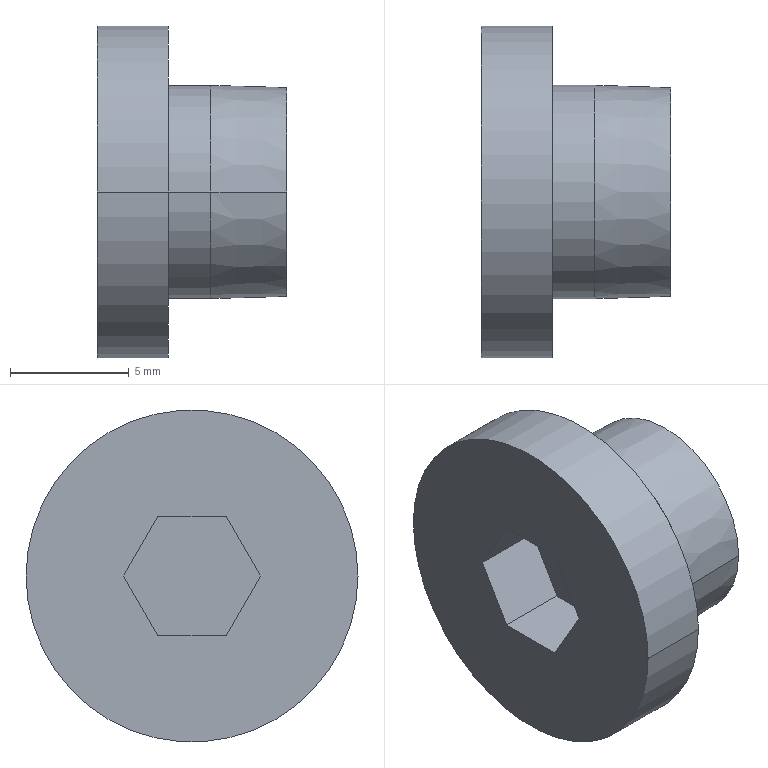Component | SolidWorks | LeverHydraulicRod22-6_Part-2 | 1 solid | 16 faces | box 8 x 14 x 14 mm | volume 710 mm3 | plane 10 | cylinder 4 | cone 2 | commonest cylinder face diameters 9 x2 14 x2
STEP:
#1=COLOUR_RGB('',0.7922,0.8196,0.9333);
#2=FILL_AREA_STYLE_COLOUR('',#1);
#3=FILL_AREA_STYLE('',(#2));
#4=SURFACE_STYLE_FILL_AREA(#3);
#5=SURFACE_SIDE_STYLE('',(#4));
#6=SURFACE_STYLE_USAGE(.BOTH.,#5);
#7=PRESENTATION_STYLE_ASSIGNMENT((#6));
#8=CARTESIAN_POINT('',(-3.607,3.128,3.307));
#9=VERTEX_POINT('',#8);
#10=CARTESIAN_POINT('',(-3.607,2.781,3.307));
#11=VERTEX_POINT('',#10);
#12=CARTESIAN_POINT('',(-3.607,2.955,3.307));
#13=DIRECTION('',(-1.,-0.,0.));
#14=DIRECTION('',(0.,-1.,0.));
#15=AXIS2_PLACEMENT_3D('',#12,#13,#14);
#16=CIRCLE('',#15,0.1732);
#17=EDGE_CURVE('',#9,#11,#16,.T.);
#18=ORIENTED_EDGE('',*,*,#17,.T.);
#19=CARTESIAN_POINT('',(-3.733,2.777,3.307));
#20=VERTEX_POINT('',#19);
#21=CARTESIAN_POINT('',(-3.745,2.777,3.307));
#22=DIRECTION('',(-0.9995,-0.0312,-0.));
#23=VECTOR('',#22,39.37);
#24=LINE('',#21,#23);
#25=EDGE_CURVE('',#11,#20,#24,.T.);
#26=ORIENTED_EDGE('',*,*,#25,.T.);
#27=CARTESIAN_POINT('',(-3.733,3.132,3.307));
#28=VERTEX_POINT('',#27);
#29=CARTESIAN_POINT('',(-3.733,2.955,3.307));
#30=DIRECTION('',(1.,0.,-0.));
#31=DIRECTION('',(0.,1.,0.));
#32=AXIS2_PLACEMENT_3D('',#29,#30,#31);
#33=CIRCLE('',#32,0.1772);
#34=EDGE_CURVE('',#20,#28,#33,.T.);
#35=ORIENTED_EDGE('',*,*,#34,.T.);
#36=CARTESIAN_POINT('',(-3.745,3.132,3.307));
#37=DIRECTION('',(-0.9995,0.0312,0.));
#38=VECTOR('',#37,39.37);
#39=LINE('',#36,#38);
#40=EDGE_CURVE('',#9,#28,#39,.T.);
#41=ORIENTED_EDGE('',*,*,#40,.F.);
#42=EDGE_LOOP('',(#18,#26,#35,#41));
#43=FACE_OUTER_BOUND('',#42,.T.);
#44=CARTESIAN_POINT('',(-3.745,2.955,3.307));
#45=DIRECTION('',(-1.,-0.,0.));
#46=DIRECTION('',(0.,1.,0.));
#47=AXIS2_PLACEMENT_3D('',#44,#45,#46);
#48=CONICAL_SURFACE('',#47,0.1775,0.03121);
#49=ADVANCED_FACE('',(#43),#48,.T.);
#50=ORIENTED_EDGE('',*,*,#34,.F.);
#51=CARTESIAN_POINT('',(-3.804,2.777,3.307));
#52=VERTEX_POINT('',#51);
#53=CARTESIAN_POINT('',(-3.607,2.777,3.307));
#54=DIRECTION('',(-1.,-0.,0.));
#55=VECTOR('',#54,39.37);
#56=LINE('',#53,#55);
#57=EDGE_CURVE('',#20,#52,#56,.T.);
#58=ORIENTED_EDGE('',*,*,#57,.T.);
#59=CARTESIAN_POINT('',(-3.804,3.132,3.307));
#60=VERTEX_POINT('',#59);
#61=CARTESIAN_POINT('',(-3.804,2.955,3.307));
#62=DIRECTION('',(1.,0.,-0.));
#63=DIRECTION('',(0.,1.,0.));
#64=AXIS2_PLACEMENT_3D('',#61,#62,#63);
#65=CIRCLE('',#64,0.1772);
#66=EDGE_CURVE('',#52,#60,#65,.T.);
#67=ORIENTED_EDGE('',*,*,#66,.T.);
#68=CARTESIAN_POINT('',(-3.607,3.132,3.307));
#69=DIRECTION('',(-1.,-0.,0.));
#70=VECTOR('',#69,39.37);
#71=LINE('',#68,#70);
#72=EDGE_CURVE('',#28,#60,#71,.T.);
#73=ORIENTED_EDGE('',*,*,#72,.F.);
#74=EDGE_LOOP('',(#50,#58,#67,#73));
#75=FACE_OUTER_BOUND('',#74,.T.);
#76=CARTESIAN_POINT('',(-3.607,2.955,3.307));
#77=DIRECTION('',(-1.,-0.,0.));
#78=DIRECTION('',(0.,1.,0.));
#79=AXIS2_PLACEMENT_3D('',#76,#77,#78);
#80=CYLINDRICAL_SURFACE('',#79,0.1772);
#81=ADVANCED_FACE('',(#75),#80,.T.);
#82=CARTESIAN_POINT('',(-3.922,3.23,3.307));
#83=VERTEX_POINT('',#82);
#84=CARTESIAN_POINT('',(-3.922,2.679,3.307));
#85=VERTEX_POINT('',#84);
#86=CARTESIAN_POINT('',(-3.922,2.955,3.307));
#87=DIRECTION('',(-1.,-0.,0.));
#88=DIRECTION('',(0.,1.,0.));
#89=AXIS2_PLACEMENT_3D('',#86,#87,#88);
#90=CIRCLE('',#89,0.2756);
#91=EDGE_CURVE('',#83,#85,#90,.T.);
#92=ORIENTED_EDGE('',*,*,#91,.F.);
#93=CARTESIAN_POINT('',(-3.804,3.23,3.307));
#94=VERTEX_POINT('',#93);
#95=CARTESIAN_POINT('',(-3.922,3.23,3.307));
#96=DIRECTION('',(1.,0.,-0.));
#97=VECTOR('',#96,39.37);
#98=LINE('',#95,#97);
#99=EDGE_CURVE('',#83,#94,#98,.T.);
#100=ORIENTED_EDGE('',*,*,#99,.T.);
#101=CARTESIAN_POINT('',(-3.804,2.679,3.307));
#102=VERTEX_POINT('',#101);
#103=CARTESIAN_POINT('',(-3.804,2.955,3.307));
#104=DIRECTION('',(-1.,-0.,0.));
#105=DIRECTION('',(0.,1.,0.));
#106=AXIS2_PLACEMENT_3D('',#103,#104,#105);
#107=CIRCLE('',#106,0.2756);
#108=EDGE_CURVE('',#94,#102,#107,.T.);
#109=ORIENTED_EDGE('',*,*,#108,.T.);
#110=CARTESIAN_POINT('',(-3.922,2.679,3.307));
#111=DIRECTION('',(1.,0.,-0.));
#112=VECTOR('',#111,39.37);
#113=LINE('',#110,#112);
#114=EDGE_CURVE('',#85,#102,#113,.T.);
#115=ORIENTED_EDGE('',*,*,#114,.F.);
#116=EDGE_LOOP('',(#92,#100,#109,#115));
#117=FACE_OUTER_BOUND('',#116,.T.);
#118=CARTESIAN_POINT('',(-3.922,2.955,3.307));
#119=DIRECTION('',(1.,0.,-0.));
#120=DIRECTION('',(0.,-1.,0.));
#121=AXIS2_PLACEMENT_3D('',#118,#119,#120);
#122=CYLINDRICAL_SURFACE('',#121,0.2756);
#123=ADVANCED_FACE('',(#117),#122,.T.);
#124=CARTESIAN_POINT('',(-3.804,2.898,3.406));
#125=VERTEX_POINT('',#124);
#126=CARTESIAN_POINT('',(-3.804,3.011,3.406));
#127=VERTEX_POINT('',#126);
#128=CARTESIAN_POINT('',(-3.804,2.898,3.406));
#129=DIRECTION('',(-0.,1.,0.));
#130=VECTOR('',#129,39.37);
#131=LINE('',#128,#130);
#132=EDGE_CURVE('',#125,#127,#131,.T.);
#133=ORIENTED_EDGE('',*,*,#132,.T.);
#134=CARTESIAN_POINT('',(-3.804,3.068,3.307));
#135=VERTEX_POINT('',#134);
#136=CARTESIAN_POINT('',(-3.804,3.011,3.406));
#137=DIRECTION('',(-0.,0.5,-0.866));
#138=VECTOR('',#137,39.37);
#139=LINE('',#136,#138);
#140=EDGE_CURVE('',#127,#135,#139,.T.);
#141=ORIENTED_EDGE('',*,*,#140,.T.);
#142=CARTESIAN_POINT('',(-3.804,3.011,3.209));
#143=VERTEX_POINT('',#142);
#144=CARTESIAN_POINT('',(-3.804,3.068,3.307));
#145=DIRECTION('',(-0.,-0.5,-0.866));
#146=VECTOR('',#145,39.37);
#147=LINE('',#144,#146);
#148=EDGE_CURVE('',#135,#143,#147,.T.);
#149=ORIENTED_EDGE('',*,*,#148,.T.);
#150=CARTESIAN_POINT('',(-3.804,2.898,3.209));
#151=VERTEX_POINT('',#150);
#152=CARTESIAN_POINT('',(-3.804,3.011,3.209));
#153=DIRECTION('',(0.,-1.,-0.));
#154=VECTOR('',#153,39.37);
#155=LINE('',#152,#154);
#156=EDGE_CURVE('',#143,#151,#155,.T.);
#157=ORIENTED_EDGE('',*,*,#156,.T.);
#158=CARTESIAN_POINT('',(-3.804,2.841,3.307));
#159=VERTEX_POINT('',#158);
#160=CARTESIAN_POINT('',(-3.804,2.898,3.209));
#161=DIRECTION('',(0.,-0.5,0.866));
#162=VECTOR('',#161,39.37);
#163=LINE('',#160,#162);
#164=EDGE_CURVE('',#151,#159,#163,.T.);
#165=ORIENTED_EDGE('',*,*,#164,.T.);
#166=CARTESIAN_POINT('',(-3.804,2.841,3.307));
#167=DIRECTION('',(0.,0.5,0.866));
#168=VECTOR('',#167,39.37);
#169=LINE('',#166,#168);
#170=EDGE_CURVE('',#159,#125,#169,.T.);
#171=ORIENTED_EDGE('',*,*,#170,.T.);
#172=EDGE_LOOP('',(#133,#141,#149,#157,#165,#171));
#173=FACE_OUTER_BOUND('',#172,.T.);
#174=CARTESIAN_POINT('',(-3.804,2.955,3.307));
#175=DIRECTION('',(-1.,-0.,0.));
#176=DIRECTION('',(-0.,1.,0.));
#177=AXIS2_PLACEMENT_3D('',#174,#175,#176);
#178=PLANE('',#177);
#179=ADVANCED_FACE('',(#173),#178,.T.);
#180=CARTESIAN_POINT('',(-3.922,3.011,3.406));
#181=VERTEX_POINT('',#180);
#182=CARTESIAN_POINT('',(-3.922,3.068,3.307));
#183=VERTEX_POINT('',#182);
#184=CARTESIAN_POINT('',(-3.922,3.011,3.406));
#185=DIRECTION('',(-0.,0.5,-0.866));
#186=VECTOR('',#185,39.37);
#187=LINE('',#184,#186);
#188=EDGE_CURVE('',#181,#183,#187,.T.);
#189=ORIENTED_EDGE('',*,*,#188,.T.);
#190=CARTESIAN_POINT('',(-3.804,3.068,3.307));
#191=DIRECTION('',(-1.,-0.,0.));
#192=VECTOR('',#191,39.37);
#193=LINE('',#190,#192);
#194=EDGE_CURVE('',#135,#183,#193,.T.);
#195=ORIENTED_EDGE('',*,*,#194,.F.);
#196=ORIENTED_EDGE('',*,*,#140,.F.);
#197=CARTESIAN_POINT('',(-3.804,3.011,3.406));
#198=DIRECTION('',(-1.,-0.,0.));
#199=VECTOR('',#198,39.37);
#200=LINE('',#197,#199);
#201=EDGE_CURVE('',#127,#181,#200,.T.);
#202=ORIENTED_EDGE('',*,*,#201,.T.);
#203=EDGE_LOOP('',(#189,#195,#196,#202));
#204=FACE_OUTER_BOUND('',#203,.T.);
#205=CARTESIAN_POINT('',(-3.804,3.011,3.406));
#206=DIRECTION('',(-0.,0.866,0.5));
#207=DIRECTION('',(1.,0.,-0.));
#208=AXIS2_PLACEMENT_3D('',#205,#206,#207);
#209=PLANE('',#208);
#210=ADVANCED_FACE('',(#204),#209,.F.);
#211=CARTESIAN_POINT('',(-3.922,3.011,3.209));
#212=VERTEX_POINT('',#211);
#213=CARTESIAN_POINT('',(-3.922,3.068,3.307));
#214=DIRECTION('',(-0.,-0.5,-0.866));
#215=VECTOR('',#214,39.37);
#216=LINE('',#213,#215);
#217=EDGE_CURVE('',#183,#212,#216,.T.);
#218=ORIENTED_EDGE('',*,*,#217,.T.);
#219=CARTESIAN_POINT('',(-3.804,3.011,3.209));
#220=DIRECTION('',(-1.,-0.,0.));
#221=VECTOR('',#220,39.37);
#222=LINE('',#219,#221);
#223=EDGE_CURVE('',#143,#212,#222,.T.);
#224=ORIENTED_EDGE('',*,*,#223,.F.);
#225=ORIENTED_EDGE('',*,*,#148,.F.);
#226=ORIENTED_EDGE('',*,*,#194,.T.);
#227=EDGE_LOOP('',(#218,#224,#225,#226));
#228=FACE_OUTER_BOUND('',#227,.T.);
#229=CARTESIAN_POINT('',(-3.804,3.068,3.307));
#230=DIRECTION('',(-0.,0.866,-0.5));
#231=DIRECTION('',(1.,0.,-0.));
#232=AXIS2_PLACEMENT_3D('',#229,#230,#231);
#233=PLANE('',#232);
#234=ADVANCED_FACE('',(#228),#233,.F.);
#235=CARTESIAN_POINT('',(-3.922,2.898,3.209));
#236=VERTEX_POINT('',#235);
#237=CARTESIAN_POINT('',(-3.922,3.011,3.209));
#238=DIRECTION('',(0.,-1.,-0.));
#239=VECTOR('',#238,39.37);
#240=LINE('',#237,#239);
#241=EDGE_CURVE('',#212,#236,#240,.T.);
#242=ORIENTED_EDGE('',*,*,#241,.T.);
#243=CARTESIAN_POINT('',(-3.804,2.898,3.209));
#244=DIRECTION('',(-1.,-0.,0.));
#245=VECTOR('',#244,39.37);
#246=LINE('',#243,#245);
#247=EDGE_CURVE('',#151,#236,#246,.T.);
#248=ORIENTED_EDGE('',*,*,#247,.F.);
#249=ORIENTED_EDGE('',*,*,#156,.F.);
#250=ORIENTED_EDGE('',*,*,#223,.T.);
#251=EDGE_LOOP('',(#242,#248,#249,#250));
#252=FACE_OUTER_BOUND('',#251,.T.);
#253=CARTESIAN_POINT('',(-3.804,3.011,3.209));
#254=DIRECTION('',(-0.,0.,-1.));
#255=DIRECTION('',(-0.,1.,0.));
#256=AXIS2_PLACEMENT_3D('',#253,#254,#255);
#257=PLANE('',#256);
#258=ADVANCED_FACE('',(#252),#257,.F.);
#259=CARTESIAN_POINT('',(-3.922,2.841,3.307));
#260=VERTEX_POINT('',#259);
#261=CARTESIAN_POINT('',(-3.922,2.898,3.209));
#262=DIRECTION('',(0.,-0.5,0.866));
#263=VECTOR('',#262,39.37);
#264=LINE('',#261,#263);
#265=EDGE_CURVE('',#236,#260,#264,.T.);
#266=ORIENTED_EDGE('',*,*,#265,.T.);
#267=CARTESIAN_POINT('',(-3.804,2.841,3.307));
#268=DIRECTION('',(-1.,-0.,0.));
#269=VECTOR('',#268,39.37);
#270=LINE('',#267,#269);
#271=EDGE_CURVE('',#159,#260,#270,.T.);
#272=ORIENTED_EDGE('',*,*,#271,.F.);
#273=ORIENTED_EDGE('',*,*,#164,.F.);
#274=ORIENTED_EDGE('',*,*,#247,.T.);
#275=EDGE_LOOP('',(#266,#272,#273,#274));
#276=FACE_OUTER_BOUND('',#275,.T.);
#277=CARTESIAN_POINT('',(-3.804,2.898,3.209));
#278=DIRECTION('',(0.,-0.866,-0.5));
#279=DIRECTION('',(-1.,-0.,0.));
#280=AXIS2_PLACEMENT_3D('',#277,#278,#279);
#281=PLANE('',#280);
#282=ADVANCED_FACE('',(#276),#281,.F.);
#283=CARTESIAN_POINT('',(-3.922,2.898,3.406));
#284=VERTEX_POINT('',#283);
#285=CARTESIAN_POINT('',(-3.922,2.841,3.307));
#286=DIRECTION('',(0.,0.5,0.866));
#287=VECTOR('',#286,39.37);
#288=LINE('',#285,#287);
#289=EDGE_CURVE('',#260,#284,#288,.T.);
#290=ORIENTED_EDGE('',*,*,#289,.T.);
#291=CARTESIAN_POINT('',(-3.804,2.898,3.406));
#292=DIRECTION('',(-1.,-0.,0.));
#293=VECTOR('',#292,39.37);
#294=LINE('',#291,#293);
#295=EDGE_CURVE('',#125,#284,#294,.T.);
#296=ORIENTED_EDGE('',*,*,#295,.F.);
#297=ORIENTED_EDGE('',*,*,#170,.F.);
#298=ORIENTED_EDGE('',*,*,#271,.T.);
#299=EDGE_LOOP('',(#290,#296,#297,#298));
#300=FACE_OUTER_BOUND('',#299,.T.);
#301=CARTESIAN_POINT('',(-3.804,2.841,3.307));
#302=DIRECTION('',(0.,-0.866,0.5));
#303=DIRECTION('',(-0.,-0.5,-0.866));
#304=AXIS2_PLACEMENT_3D('',#301,#302,#303);
#305=PLANE('',#304);
#306=ADVANCED_FACE('',(#300),#305,.F.);
#307=CARTESIAN_POINT('',(-3.922,2.898,3.406));
#308=DIRECTION('',(-0.,1.,0.));
#309=VECTOR('',#308,39.37);
#310=LINE('',#307,#309);
#311=EDGE_CURVE('',#284,#181,#310,.T.);
#312=ORIENTED_EDGE('',*,*,#311,.T.);
#313=ORIENTED_EDGE('',*,*,#201,.F.);
#314=ORIENTED_EDGE('',*,*,#132,.F.);
#315=ORIENTED_EDGE('',*,*,#295,.T.);
#316=EDGE_LOOP('',(#312,#313,#314,#315));
#317=FACE_OUTER_BOUND('',#316,.T.);
#318=CARTESIAN_POINT('',(-3.804,2.898,3.406));
#319=DIRECTION('',(0.,-0.,1.));
#320=DIRECTION('',(1.,0.,-0.));
#321=AXIS2_PLACEMENT_3D('',#318,#319,#320);
#322=PLANE('',#321);
#323=ADVANCED_FACE('',(#317),#322,.F.);
#324=ORIENTED_EDGE('',*,*,#311,.F.);
#325=ORIENTED_EDGE('',*,*,#289,.F.);
#326=ORIENTED_EDGE('',*,*,#265,.F.);
#327=ORIENTED_EDGE('',*,*,#241,.F.);
#328=ORIENTED_EDGE('',*,*,#217,.F.);
#329=ORIENTED_EDGE('',*,*,#188,.F.);
#330=EDGE_LOOP('',(#324,#325,#326,#327,#328,#329));
#331=FACE_BOUND('',#330,.T.);
#332=CARTESIAN_POINT('',(-3.922,2.955,3.307));
#333=DIRECTION('',(-1.,-0.,0.));
#334=DIRECTION('',(0.,1.,0.));
#335=AXIS2_PLACEMENT_3D('',#332,#333,#334);
#336=CIRCLE('',#335,0.2756);
#337=EDGE_CURVE('',#85,#83,#336,.T.);
#338=ORIENTED_EDGE('',*,*,#337,.T.);
#339=ORIENTED_EDGE('',*,*,#91,.T.);
#340=EDGE_LOOP('',(#338,#339));
#341=FACE_OUTER_BOUND('',#340,.T.);
#342=CARTESIAN_POINT('',(-3.922,2.955,3.307));
#343=DIRECTION('',(-1.,-0.,0.));
#344=DIRECTION('',(-0.,1.,0.));
#345=AXIS2_PLACEMENT_3D('',#342,#343,#344);
#346=PLANE('',#345);
#347=ADVANCED_FACE('',(#331,#341),#346,.T.);
#348=CARTESIAN_POINT('',(-3.804,2.955,3.307));
#349=DIRECTION('',(1.,0.,-0.));
#350=DIRECTION('',(0.,1.,0.));
#351=AXIS2_PLACEMENT_3D('',#348,#349,#350);
#352=CIRCLE('',#351,0.1772);
#353=EDGE_CURVE('',#60,#52,#352,.T.);
#354=ORIENTED_EDGE('',*,*,#353,.F.);
#355=ORIENTED_EDGE('',*,*,#66,.F.);
#356=EDGE_LOOP('',(#354,#355));
#357=FACE_BOUND('',#356,.T.);
#358=CARTESIAN_POINT('',(-3.804,2.955,3.307));
#359=DIRECTION('',(-1.,-0.,0.));
#360=DIRECTION('',(0.,1.,0.));
#361=AXIS2_PLACEMENT_3D('',#358,#359,#360);
#362=CIRCLE('',#361,0.2756);
#363=EDGE_CURVE('',#102,#94,#362,.T.);
#364=ORIENTED_EDGE('',*,*,#363,.F.);
#365=ORIENTED_EDGE('',*,*,#108,.F.);
#366=EDGE_LOOP('',(#364,#365));
#367=FACE_OUTER_BOUND('',#366,.T.);
#368=CARTESIAN_POINT('',(-3.804,2.955,3.307));
#369=DIRECTION('',(-1.,-0.,0.));
#370=DIRECTION('',(-0.,1.,0.));
#371=AXIS2_PLACEMENT_3D('',#368,#369,#370);
#372=PLANE('',#371);
#373=ADVANCED_FACE('',(#357,#367),#372,.F.);
#374=ORIENTED_EDGE('',*,*,#99,.F.);
#375=ORIENTED_EDGE('',*,*,#337,.F.);
#376=ORIENTED_EDGE('',*,*,#114,.T.);
#377=ORIENTED_EDGE('',*,*,#363,.T.);
#378=EDGE_LOOP('',(#374,#375,#376,#377));
#379=FACE_OUTER_BOUND('',#378,.T.);
#380=CARTESIAN_POINT('',(-3.922,2.955,3.307));
#381=DIRECTION('',(1.,0.,-0.));
#382=DIRECTION('',(0.,-1.,0.));
#383=AXIS2_PLACEMENT_3D('',#380,#381,#382);
#384=CYLINDRICAL_SURFACE('',#383,0.2756);
#385=ADVANCED_FACE('',(#379),#384,.T.);
#386=ORIENTED_EDGE('',*,*,#57,.F.);
#387=CARTESIAN_POINT('',(-3.733,2.955,3.307));
#388=DIRECTION('',(1.,0.,-0.));
#389=DIRECTION('',(0.,1.,0.));
#390=AXIS2_PLACEMENT_3D('',#387,#388,#389);
#391=CIRCLE('',#390,0.1772);
#392=EDGE_CURVE('',#28,#20,#391,.T.);
#393=ORIENTED_EDGE('',*,*,#392,.F.);
#394=ORIENTED_EDGE('',*,*,#72,.T.);
#395=ORIENTED_EDGE('',*,*,#353,.T.);
#396=EDGE_LOOP('',(#386,#393,#394,#395));
#397=FACE_OUTER_BOUND('',#396,.T.);
#398=CARTESIAN_POINT('',(-3.607,2.955,3.307));
#399=DIRECTION('',(-1.,-0.,0.));
#400=DIRECTION('',(0.,1.,0.));
#401=AXIS2_PLACEMENT_3D('',#398,#399,#400);
#402=CYLINDRICAL_SURFACE('',#401,0.1772);
#403=ADVANCED_FACE('',(#397),#402,.T.);
#404=ORIENTED_EDGE('',*,*,#25,.F.);
#405=CARTESIAN_POINT('',(-3.607,2.955,3.307));
#406=DIRECTION('',(-1.,-0.,0.));
#407=DIRECTION('',(0.,-1.,0.));
#408=AXIS2_PLACEMENT_3D('',#405,#406,#407);
#409=CIRCLE('',#408,0.1732);
#410=EDGE_CURVE('',#11,#9,#409,.T.);
#411=ORIENTED_EDGE('',*,*,#410,.T.);
#412=ORIENTED_EDGE('',*,*,#40,.T.);
#413=ORIENTED_EDGE('',*,*,#392,.T.);
#414=EDGE_LOOP('',(#404,#411,#412,#413));
#415=FACE_OUTER_BOUND('',#414,.T.);
#416=CARTESIAN_POINT('',(-3.745,2.955,3.307));
#417=DIRECTION('',(-1.,-0.,0.));
#418=DIRECTION('',(0.,1.,0.));
#419=AXIS2_PLACEMENT_3D('',#416,#417,#418);
#420=CONICAL_SURFACE('',#419,0.1775,0.03121);
#421=ADVANCED_FACE('',(#415),#420,.T.);
#422=ORIENTED_EDGE('',*,*,#17,.F.);
#423=ORIENTED_EDGE('',*,*,#410,.F.);
#424=EDGE_LOOP('',(#422,#423));
#425=FACE_OUTER_BOUND('',#424,.T.);
#426=CARTESIAN_POINT('',(-3.607,2.955,3.307));
#427=DIRECTION('',(1.,0.,-0.));
#428=DIRECTION('',(0.,-0.,1.));
#429=AXIS2_PLACEMENT_3D('',#426,#427,#428);
#430=PLANE('',#429);
#431=ADVANCED_FACE('',(#425),#430,.T.);
#432=CLOSED_SHELL('',(#49,#81,#123,#179,#210,#234,#258,#282,#306,#323,#347,#373,#385,#403,#421,#431));
#433=MANIFOLD_SOLID_BREP('',#432);
#434=STYLED_ITEM('',(#7),#433);
#435=(LENGTH_UNIT()NAMED_UNIT(*)SI_UNIT($,.METRE.));
#436=LENGTH_MEASURE_WITH_UNIT(LENGTH_MEASURE(0.0254),#435);
#437=DIMENSIONAL_EXPONENTS(1.,0.,0.,0.,0.,0.,0.);
#438=(CONVERSION_BASED_UNIT('',#436)LENGTH_UNIT()NAMED_UNIT(#437));
#439=UNCERTAINTY_MEASURE_WITH_UNIT(LENGTH_MEASURE(0.00001),#438,'','');
#440=(NAMED_UNIT(*)PLANE_ANGLE_UNIT()SI_UNIT($,.RADIAN.));
#441=(NAMED_UNIT(*)SI_UNIT($,.STERADIAN.)SOLID_ANGLE_UNIT());
#442=(GEOMETRIC_REPRESENTATION_CONTEXT(3)GLOBAL_UNCERTAINTY_ASSIGNED_CONTEXT((#439))GLOBAL_UNIT_ASSIGNED_CONTEXT((#438,#440,#441))REPRESENTATION_CONTEXT('',''));
#443=MECHANICAL_DESIGN_GEOMETRIC_PRESENTATION_REPRESENTATION('',(#434),#442);
#444=CARTESIAN_POINT('',(0.,0.,0.));
#445=DIRECTION('',(0.,0.,1.));
#446=DIRECTION('',(1.,0.,0.));
#447=AXIS2_PLACEMENT_3D('',#444,#445,#446);
#448=(LENGTH_UNIT()NAMED_UNIT(*)SI_UNIT($,.METRE.));
#449=LENGTH_MEASURE_WITH_UNIT(LENGTH_MEASURE(0.0254),#448);
#450=DIMENSIONAL_EXPONENTS(1.,0.,0.,0.,0.,0.,0.);
#451=(CONVERSION_BASED_UNIT('',#449)LENGTH_UNIT()NAMED_UNIT(#450));
#452=UNCERTAINTY_MEASURE_WITH_UNIT(LENGTH_MEASURE(0.00001),#451,'','');
#453=(NAMED_UNIT(*)PLANE_ANGLE_UNIT()SI_UNIT($,.RADIAN.));
#454=(NAMED_UNIT(*)SI_UNIT($,.STERADIAN.)SOLID_ANGLE_UNIT());
#455=(GEOMETRIC_REPRESENTATION_CONTEXT(3)GLOBAL_UNCERTAINTY_ASSIGNED_CONTEXT((#452))GLOBAL_UNIT_ASSIGNED_CONTEXT((#451,#453,#454))REPRESENTATION_CONTEXT('',''));
#456=ADVANCED_BREP_SHAPE_REPRESENTATION('',(#433,#447),#455);
#457=PRESENTATION_LAYER_ASSIGNMENT('','',(#434));